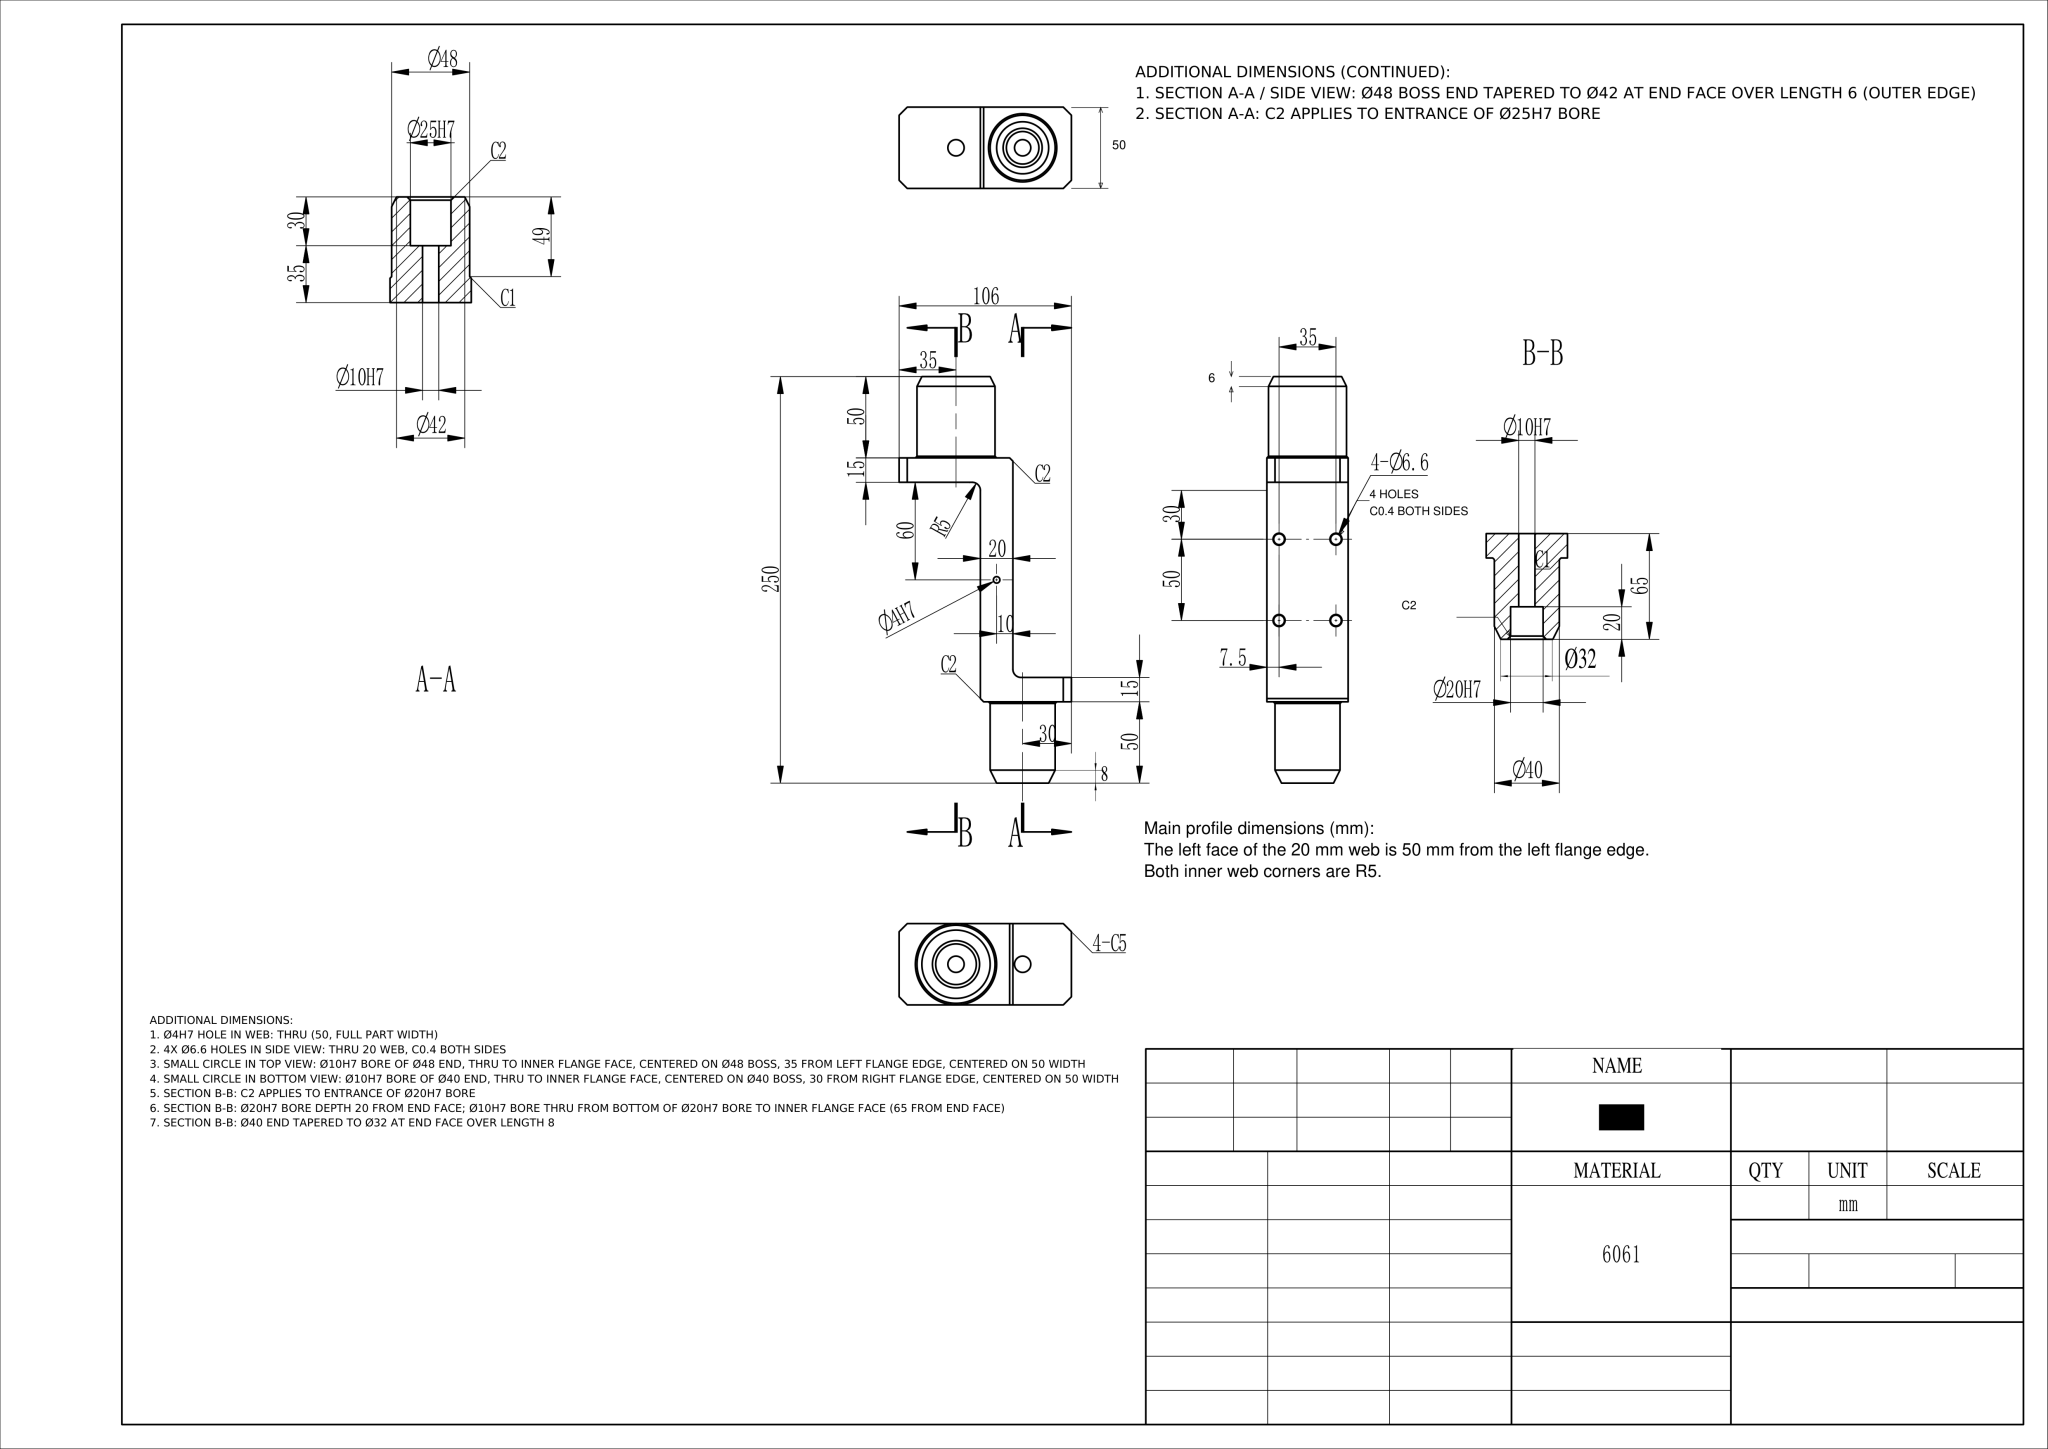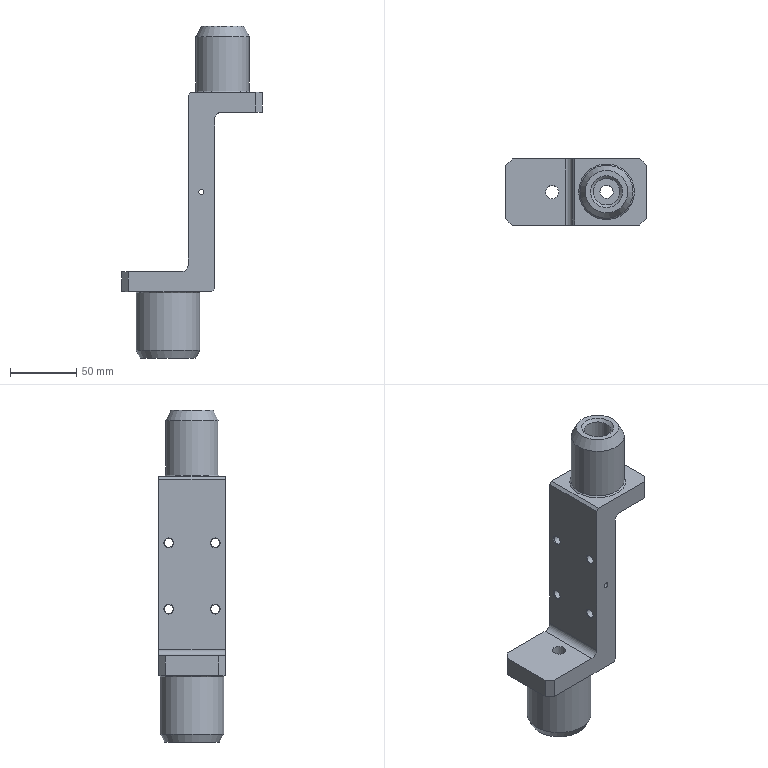Part | NX | mm | 1 solid | 48 faces | box 106 x 50 x 250 mm | volume 333376 mm3 | plane 21 | cone 14 | cylinder 13 | commonest cylinder face diameters 10 x4 6.6 x4 40 x1 48 x1 20 x1 25 x1 4 x1